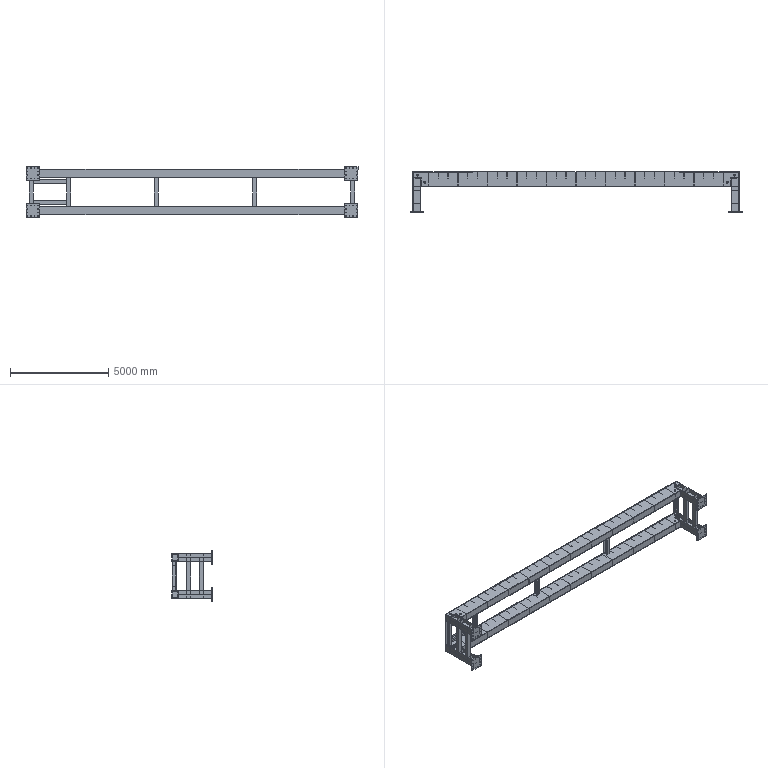Assembly | SolidWorks | mm | 129 component files | 129 solids | 1298 faces | box 16880 x 2070 x 2580 mm | volume 955570944 mm3 | plane 894 | cylinder 404 | commonest cylinder face diameters 25 x320 100 x32 20 x16 10 x16 3440371.25 x10 3440351.25 x6 3432081.25 x4
Bill of materials:
200 x 200 x 5 | 4 | Plain Carbon Steel | Long straight hollow square tube with thin walls and rounded outer and inner corners.
BlockingPlate | 4 | Plain Carbon Steel | Thin flat rectangular plate, slightly taller than it is wide, with no features.
ColumnRibPlate | 24 | Plain Carbon Steel | Flat rectangular plate, about twice as long as it is high, with no features.
ConnectingPlate | 4 | Plain Carbon Steel | Flat rectangular plate with six round through-holes, laid out as two rows of three near the top and bottom edges.
Flange25 | 4 | Plain Carbon Steel | Flat, nearly square plate with twelve small round through-holes evenly spaced around its edges, leaving the centre clear.
I-Beam | 4 | Plain Carbon Steel | Short H/I-section beam segment with two parallel flanges joined by a central web. One flange has six small round holes near one end.
I-Beam200 | 5 | Plain Carbon Steel | Long straight I/H-section member: two wide flanges joined by a thin central web, with no holes visible.
I-Beam200-1905 | 2 | Plain Carbon Steel | Long H-section member with two tall parallel flanges and a thin connecting web. The web runs slightly past the flange ends at both ends.
LowerCover | 2 | Plain Carbon Steel | Long, slender, straight flat bar or strip with a thin rectangular cross-section.
RibPlate | 22 | Plain Carbon Steel | Very thin flat rectangular sheet, about 2:1, with no features.
RibPlate2 | 40 | Plain Carbon Steel | Very thin, nearly square flat sheet with no features.
SidePlate | 4 | Plain Carbon Steel | Long, very thin flat strip with stepped ends. Each end has an offset narrower tab, and each end has two small round holes, one in the tab and one in the main body.
SmallFlange20 | 4 | Plain Carbon Steel | Flat square plate with constant thickness and eight round through-holes. The holes sit on a 3x3 grid with the centre position left empty, so they form a square ring set in from the edges.
SmallFlange25 | 4 | Plain Carbon Steel | Flat square plate with eight round through-holes on a 3x3 grid with the centre position left empty. Its layout matches unnamed part, but its edge appears a little thicker in the render.
UpperCover | 2 | Plain Carbon Steel | Very thin, flat, long rectangular strip or sheet with no visible holes or other features.
Mates:
1. coincident | Flange25-1 face at (664.937, 1194.803, 1855.287) dir (0, 1, 0) | I-Beam-1 face at (464.937, 1194.803, 2055.287) dir (0, -1, 0)
2. distance | I-Beam-1 face at (464.937, 2874.803, 2055.287) dir (-1, 0, 0) | Flange25-1 face at (319.937, 1169.803, 1510.287) dir (-1, 0, 0)
3. distance | I-Beam-1 face at (485.937, 2874.803, 2055.287) dir (0, 0, 1) | Flange25-1 face at (319.937, 1169.803, 2200.287) dir (0, 0, 1)
4. coincident | I-Beam-1 face at (464.937, 2874.803, 2055.287) dir (0, 1, 0) | SmallFlange25-1 face at (664.937, 2874.803, 1855.287) dir (0, -1, 0)
5. coincident | I-Beam-1 face at (464.937, 2874.803, 2055.287) dir (-1, 0, 0) | SmallFlange25-1 face at (464.937, 2874.803, 1655.287) dir (-1, 0, 0)
6. coincident | I-Beam-1 face at (464.937, 2874.803, 1655.287) dir (0, 0, -1) | SmallFlange25-1 face at (464.937, 2874.803, 1655.287) dir (0, 0, -1)
7. coincident | SmallFlange25-1 face at (664.937, 2899.803, 1855.287) dir (0, 1, 0) | SmallFlange20-1 face at (664.937, 2899.803, 1855.287) dir (0, -1, 0)
8. coincident | SmallFlange25-1 face at (464.937, 2874.803, 1655.287) dir (-1, 0, 0) | SmallFlange20-1 face at (464.937, 2899.803, 1655.287) dir (-1, 0, 0)
9. coincident | SmallFlange25-1 face at (464.937, 2874.803, 2055.287) dir (0, 0, 1) | SmallFlange20-1 face at (464.937, 2899.803, 2055.287) dir (0, 0, 1)
10. distance | SmallFlange20-1 face at (464.937, 2899.803, 1655.287) dir (-1, 0, 0) | SidePlate-1 face at (474.937, 3209.803, 2024.287) dir (-1, 0, 0)
11. coincident | SmallFlange20-1 face at (664.937, 2919.803, 1855.287) dir (0, 1, 0) | SidePlate-1 face at (474.937, 2919.803, 2024.287) dir (0, -1, 0)
12. coincident | SmallFlange20-1 face at (664.937, 2919.803, 1855.287) dir (0, 1, 0) | BlockingPlate-1 face at (464.937, 2919.803, 2055.287) dir (0, -1, 0)
13. coincident | SmallFlange20-1 face at (464.937, 2899.803, 1655.287) dir (-1, 0, 0) | BlockingPlate-1 face at (464.937, 3064.803, 1855.287) dir (-1, 0, 0)
14. coincident | SmallFlange20-1 face at (464.937, 2899.803, 1655.287) dir (0, 0, -1) | BlockingPlate-1 face at (464.937, 3209.803, 1655.287) dir (0, 0, -1)
15. coincident | SidePlate-1 face at (17044.937, 2919.803, 2024.287) dir (0, -1, 0) | ConnectingPlate-1 face at (16634.937, 2919.803, 2055.287) dir (0, 1, 0)
16. coincident | I-Beam-1 face at (864.937, 2874.803, 1655.287) dir (1, 0, 0) | ConnectingPlate-5 face at (864.937, 2699.803, 1855.287) dir (-1, 0, 0)
17. coincident | SidePlate-1 face at (474.937, 2919.803, 2024.287) dir (0, -1, 0) | ConnectingPlate-5 face at (884.937, 2919.803, 1655.287) dir (0, 1, 0)
18. coincident | SmallFlange25-1 face at (464.937, 2874.803, 2055.287) dir (0, 0, 1) | ConnectingPlate-5 face at (884.937, 2919.803, 2055.287) dir (0, 0, 1)
19. coincident | SidePlate-2 face at (8759.937, -1712810.822, 1686.287) dir (0, 0, 1) | RibPlate-2 face at (1262.937, 2499.803, 1686.287) dir (0, 0, -1)
20. distance | BlockingPlate-1 face at (464.937, 3064.803, 1855.287) dir (-1, 0, 0) | RibPlate-2 face at (1256.937, 2854.803, 1855.287) dir (-1, 0, 0)
21. coincident | BlockingPlate-1 face at (464.937, 3209.803, 2055.287) dir (0, 1, 0) | RibPlate-2 face at (1262.937, 3209.803, 1686.287) dir (0, 1, 0)
22. distance | RibPlate2-1 face at (1756.937, 3059.803, 1855.287) dir (-1, 0, 0) | RibPlate-2 face at (1262.937, 2854.803, 1855.287) dir (1, 0, 0)
23. coincident | SidePlate-2 face at (8759.937, -1712810.822, 1686.287) dir (0, 0, 1) | RibPlate2-1 face at (1762.937, 2909.803, 1686.287) dir (0, 0, -1)
24. coincident | RibPlate-2 face at (1262.937, 3209.803, 1686.287) dir (0, 1, 0) | RibPlate2-1 face at (1762.937, 3209.803, 1686.287) dir (0, 1, 0)
25. coincident | BlockingPlate-1 face at (464.937, 3064.803, 1855.287) dir (-1, 0, 0) | UpperCover-1 edge at (464.937, 3219.803, 2055.287) dir (0, 0, -1)
26. coincident | BlockingPlate-1 face at (464.937, 3209.803, 2055.287) dir (0, 0, 1) | UpperCover-1 face at (8759.937, -1716945.822, 2055.287) dir (0, 0, 1)
27. coincident | BlockingPlate-5 face at (17044.937, 3209.803, 2055.287) dir (0, 1, 0) | UpperCover-1 edge at (17054.889, 3209.803, 2055.287) dir (0, 0, -1)
28. coincident | BlockingPlate-1 face at (464.937, 3209.803, 2055.287) dir (0, 1, 0) | UpperCover-1 edge at (464.985, 3209.803, 2055.287) dir (0, 0, -1)
29. coincident | BlockingPlate-5 face at (17054.937, 3064.803, 1855.287) dir (1, 0, 0) | SmallFlange20-5 face at (17054.937, 2899.803, 2055.287) dir (1, 0, 0)
30. coincident | BlockingPlate-5 face at (17044.937, 3209.803, 2055.287) dir (0, 0, 1) | SmallFlange20-5 face at (17054.937, 2899.803, 2055.287) dir (0, 0, 1)
31. coincident | BlockingPlate-5 face at (17044.937, 2919.803, 2055.287) dir (0, -1, 0) | SmallFlange20-5 face at (16854.937, 2919.803, 1855.287) dir (0, 1, 0)
32. coincident | ConnectingPlate-1 face at (16634.937, 2919.803, 2055.287) dir (0, 0, 1) | I-Beam-5 face at (16675.937, 2874.803, 2055.287) dir (0, 0, 1)
33. coincident | ConnectingPlate-1 face at (16654.937, 2699.803, 1855.287) dir (1, 0, 0) | I-Beam-5 face at (16654.937, 2874.803, 2055.287) dir (-1, 0, 0)
34. coincident | ConnectingPlate-1 face at (16634.937, 2919.803, 2055.287) dir (0, 1, 0) | SmallFlange20-5 face at (16854.937, 2919.803, 1855.287) dir (0, 1, 0)
35. coincident | SidePlate-1 face at (17044.937, 2919.803, 2024.287) dir (1, 0, 0) | BlockingPlate-5 face at (17044.937, 3064.803, 1855.287) dir (-1, 0, 0)
36. coincident | BlockingPlate-1 face at (464.937, 3209.803, 2055.287) dir (0, 0, 1) | BlockingPlate-5 face at (17044.937, 3209.803, 2055.287) dir (0, 0, 1)
37. concentric | SidePlate-1 face at (8759.937, -1717685.822, 2024.287) dir (0, 0, 1) r 1720185.625 | LowerCover-1 face at (8759.937, -1717685.822, 1655.287) dir (0, 0, 1) r 1720185.625
38. coincident | ConnectingPlate-5 face at (884.937, 2919.803, 2055.287) dir (0, 0, 1) | LowerCover-1 face at (8759.937, -1717685.822, 2055.287) dir (0, 0, 1)
39. distance | I-Beam-5 face at (16654.937, 2874.803, 2055.287) dir (-1, 0, 0) | LowerCover-1 edge at (16652.437, 2471.697, 1655.287) dir (0, 0, 1)
40. coincident | LowerCover-1 edge at (867.437, 2471.697, 2055.287) dir (0, 0, -1) | ColumnRibPlate-1 face at (664.937, 2471.697, 1959.287) dir (0, -1, 0)
41. coincident | I-Beam-1 face at (843.937, 2874.803, 1863.287) dir (0, 0, 1) | ColumnRibPlate-1 face at (485.937, 2471.697, 1863.287) dir (0, 0, -1)
42. coincident | I-Beam-1 face at (485.937, 2874.803, 1863.287) dir (1, 0, 0) | ColumnRibPlate-1 face at (485.937, 2471.697, 1863.287) dir (-1, 0, 0)
43. parallel | SmallFlange20-1 face at (664.937, 2919.803, 1855.287) dir (0, 1, 0) | ColumnRibPlate-1 face at (664.937, 2481.697, 1959.287) dir (0, 1, 0)
44. distance | Flange25-1 face at (664.937, 1194.803, 1855.287) dir (0, 1, 0) | ColumnRibPlate-23 face at (664.937, 1614.803, 1959.287) dir (0, -1, 0)
45. coincident | I-Beam-1 face at (843.937, 2874.803, 2055.287) dir (-1, 0, 0) | ColumnRibPlate-23 face at (843.937, 1614.803, 1863.287) dir (1, 0, 0)
46. coincident | I-Beam-1 face at (843.937, 2874.803, 1863.287) dir (0, 0, 1) | ColumnRibPlate-23 face at (485.937, 1614.803, 1863.287) dir (0, 0, -1)
47. coincident | I-Beam-1 face at (843.937, 2874.803, 1863.287) dir (0, 0, 1) | 200 x 200 x 5-1 face at (495.937, 2281.697, 1863.287) dir (0, 0, -1)
48. coincident | ColumnRibPlate-4 face at (664.937, 2271.697, 1959.287) dir (0, 1, 0) | 200 x 200 x 5-1 face at (495.937, 2271.697, 3737.287) dir (0, -1, 0)
49. coincident | I-Beam-1 face at (485.937, 2874.803, 1863.287) dir (1, 0, 0) | 200 x 200 x 5-1 face at (485.937, 2281.697, 3737.287) dir (-1, 0, 0)
50. coincident | SidePlate-4 face at (8759.937, -1712810.822, 3570.287) dir (0, 0, -1) | I-Beam200-1 face at (674.937, 3009.803, 3570.287) dir (0, 0, 1)
51. coincident | BlockingPlate-4 face at (474.937, 3064.803, 3745.287) dir (1, 0, 0) | I-Beam200-1 face at (474.937, 3197.803, 3570.287) dir (-1, 0, 0)
52. coincident | BlockingPlate-1 edge at (464.937, 3209.803, 2055.287) dir (1, 0, 0) | I-Beam200-1 face at (474.937, 3209.803, 3570.287) dir (0, 1, 0)
53. coincident | I-Beam200-2 face at (2399.937, 3209.803, 3570.287) dir (0, 1, 0) | I-Beam200-1905-1 face at (584.937, 3209.803, 3220.287) dir (0, 1, 0)
54. coincident | I-Beam200-2 face at (2399.937, 3197.803, 3570.287) dir (-1, 0, 0) | I-Beam200-1905-1 face at (2399.937, 3197.803, 3220.287) dir (1, 0, 0)
55. distance | I-Beam200-1905-1 face at (584.937, 3197.803, 3220.287) dir (0, 0, -1) | I-Beam200-2 edge at (2399.937, 3209.803, 2800.287) dir (1, 0, 0)